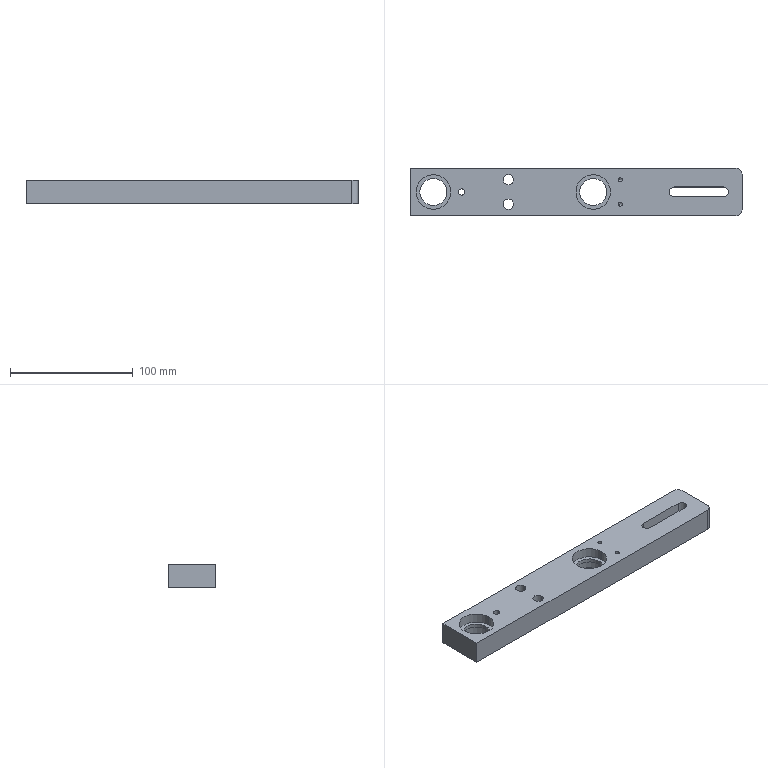Component | SolidWorks | TAR-02-019PaperCollectionMotorPlate-1 | 1 solid | 57 faces | box 270 x 39 x 19 mm | volume 165881 mm3 | cylinder 35 | plane 14 | cone 8 | commonest cylinder face diameters 28 x8 4.2 x4 13.5 x4 8.5 x4 3.3 x4 22 x4 8.1 x3 5 x2
build123d program:
from build123d import *

# Parameters (mm, degrees)
SKETCH1_R                                           = 11
BOSS_EXTRUDE1_DEPTH                                 = 19
M4_TAPPED_HOLE1_D                                   = 3.3
M4_TAPPED_HOLE1_DEPTH                               = 15
M4_TAPPED_HOLE1_TIP                                 = 0.9914
M6_TAPPED_HOLE1_D                                   = 5
CYLINDRICAL_COUNTERSUNK_HOLE_FOR_M6_HEX_D           = 8.5
CYLINDRICAL_COUNTERSUNK_HOLE_FOR_M6_HEX_CBORE_D     = 13.5
CYLINDRICAL_COUNTERSUNK_HOLE_FOR_M6_HEX_CBORE_DEPTH = 8.5
M5_TAPPED_HOLE2_D                                   = 4.2
M5_TAPPED_HOLE2_DEPTH                               = 21.4
M5_TAPPED_HOLE2_TIP                                 = 1.262
SKETCH11_R                                          = 14
CUT_EXTRUDE1_DEPTH                                  = 8
CUT_EXTRUDE2_START                                  = -8
SKETCH12_R                                          = 14
CUT_EXTRUDE2_DEPTH                                  = 8


with BuildPart() as part:
    # Sketch1 → Boss-Extrude1 (new body)
    with BuildSketch(Plane.XY):
        with BuildLine():
            Line((130, -19.5), (-135, -19.5))
            Line((-135, -19.5), (-135, 19.5))
            Line((-135, 19.5), (130, 19.5))
            ThreePointArc((130, 19.5), (133.536, 18.036), (135, 14.5))
            Line((135, 14.5), (135, -14.5))
            ThreePointArc((135, -14.5), (133.536, -18.036), (130, -19.5))
        make_face()
        with Locations((-116, 0)):
            Circle(SKETCH1_R, mode=Mode.SUBTRACT)
        with Locations((14, 0)):
            Circle(SKETCH1_R, mode=Mode.SUBTRACT)
        with BuildLine():
            Line((80, 4.05), (120, 4.05))
            ThreePointArc((120, 4.05), (124.05, 0), (120, -4.05))
            Line((120, -4.05), (80, -4.05))
            ThreePointArc((80, -4.05), (75.95, 0), (80, 4.05))
        make_face(mode=Mode.SUBTRACT)
    extrude(amount=BOSS_EXTRUDE1_DEPTH)

    # M4 Tapped Hole1
    with Locations(Plane(origin=(36, 10, 19), x_dir=(1, 0, 0), z_dir=(0, 0, 1))):
        with Locations((0, 0), (0, -20)):
            Hole(M4_TAPPED_HOLE1_D / 2, depth=M4_TAPPED_HOLE1_DEPTH)
            with Locations((0, 0, -(M4_TAPPED_HOLE1_DEPTH + M4_TAPPED_HOLE1_TIP / 2))):  # 118° drill point
                Cone(0, M4_TAPPED_HOLE1_D / 2, M4_TAPPED_HOLE1_TIP, mode=Mode.SUBTRACT)

    # M6 Tapped Hole1 (through all)
    with Locations(Plane(origin=(-93, 0, 19), x_dir=(1, 0, 0), z_dir=(0, 0, 1))):
        with Locations((0, 0)):
            Hole(M6_TAPPED_HOLE1_D / 2)

    # Cylindrical Countersunk Hole for M6 Hex (through all)
    with Locations(Plane(origin=(-55, 10, 0), x_dir=(-1, 0, 0), z_dir=(0, 0, -1))):
        with Locations((0, 0), (0, -20)):
            CounterBoreHole(CYLINDRICAL_COUNTERSUNK_HOLE_FOR_M6_HEX_D / 2, CYLINDRICAL_COUNTERSUNK_HOLE_FOR_M6_HEX_CBORE_D / 2, CYLINDRICAL_COUNTERSUNK_HOLE_FOR_M6_HEX_CBORE_DEPTH)

    # M5 Tapped Hole2
    with Locations(Plane(origin=(-29, 19.5, 9.5), x_dir=(1, 0, 0), z_dir=(0, 1, 0))):
        with Locations((0, 0), (15, 0)):
            Hole(M5_TAPPED_HOLE2_D / 2, depth=M5_TAPPED_HOLE2_DEPTH)
            with Locations((0, 0, -(M5_TAPPED_HOLE2_DEPTH + M5_TAPPED_HOLE2_TIP / 2))):  # 118° drill point
                Cone(0, M5_TAPPED_HOLE2_D / 2, M5_TAPPED_HOLE2_TIP, mode=Mode.SUBTRACT)

    # Sketch11 → Cut-Extrude1 (cut)
    with BuildSketch(Plane(origin=(0, 0, 0), x_dir=(-1, 0, 0), z_dir=(0, 0, -1))):
        with Locations((116, 0)):
            Circle(SKETCH11_R)
        with Locations((-14, 0)):
            Circle(SKETCH11_R)
    extrude(amount=-CUT_EXTRUDE1_DEPTH, mode=Mode.SUBTRACT)

    # Sketch12 → Cut-Extrude2 (cut)
    with BuildSketch(Plane.XY.offset(19).offset(CUT_EXTRUDE2_START)):
        with Locations(Location((14, 0, 0), (0, 0, 180))):
            Circle(SKETCH12_R)
        with Locations(Location((-116, 0, 0), (0, 0, 180))):
            Circle(SKETCH12_R)
    extrude(amount=CUT_EXTRUDE2_DEPTH, mode=Mode.SUBTRACT)


solid = part.part

# Placed as in the assembly
solid = solid.moved(Location((0.609, 9.288, -9.5), (0, 0, 0)))